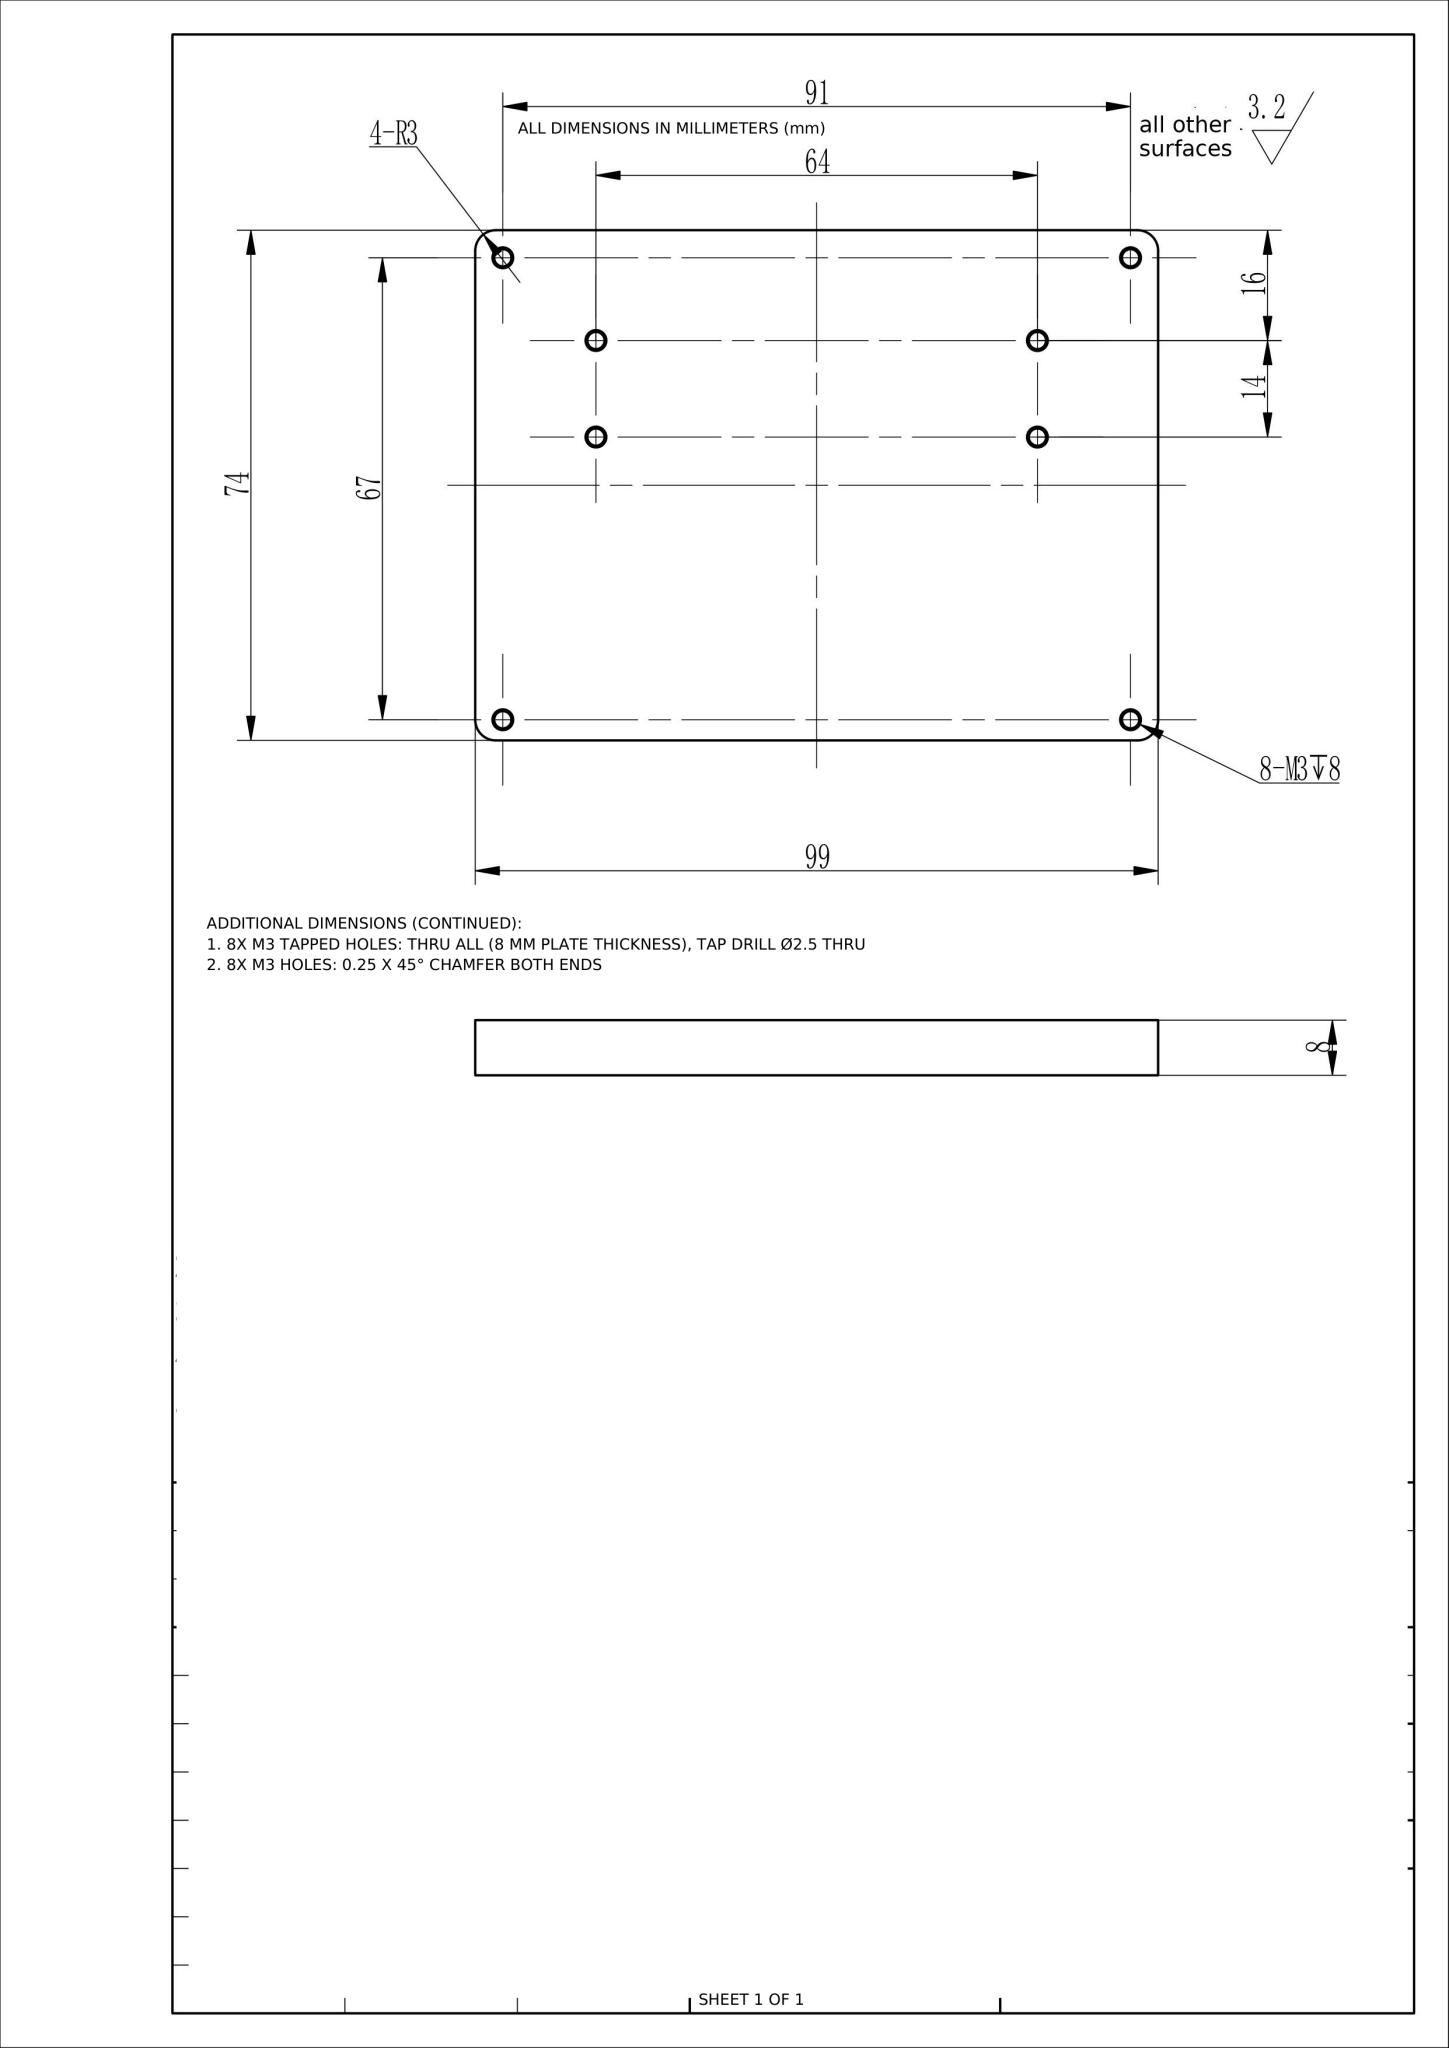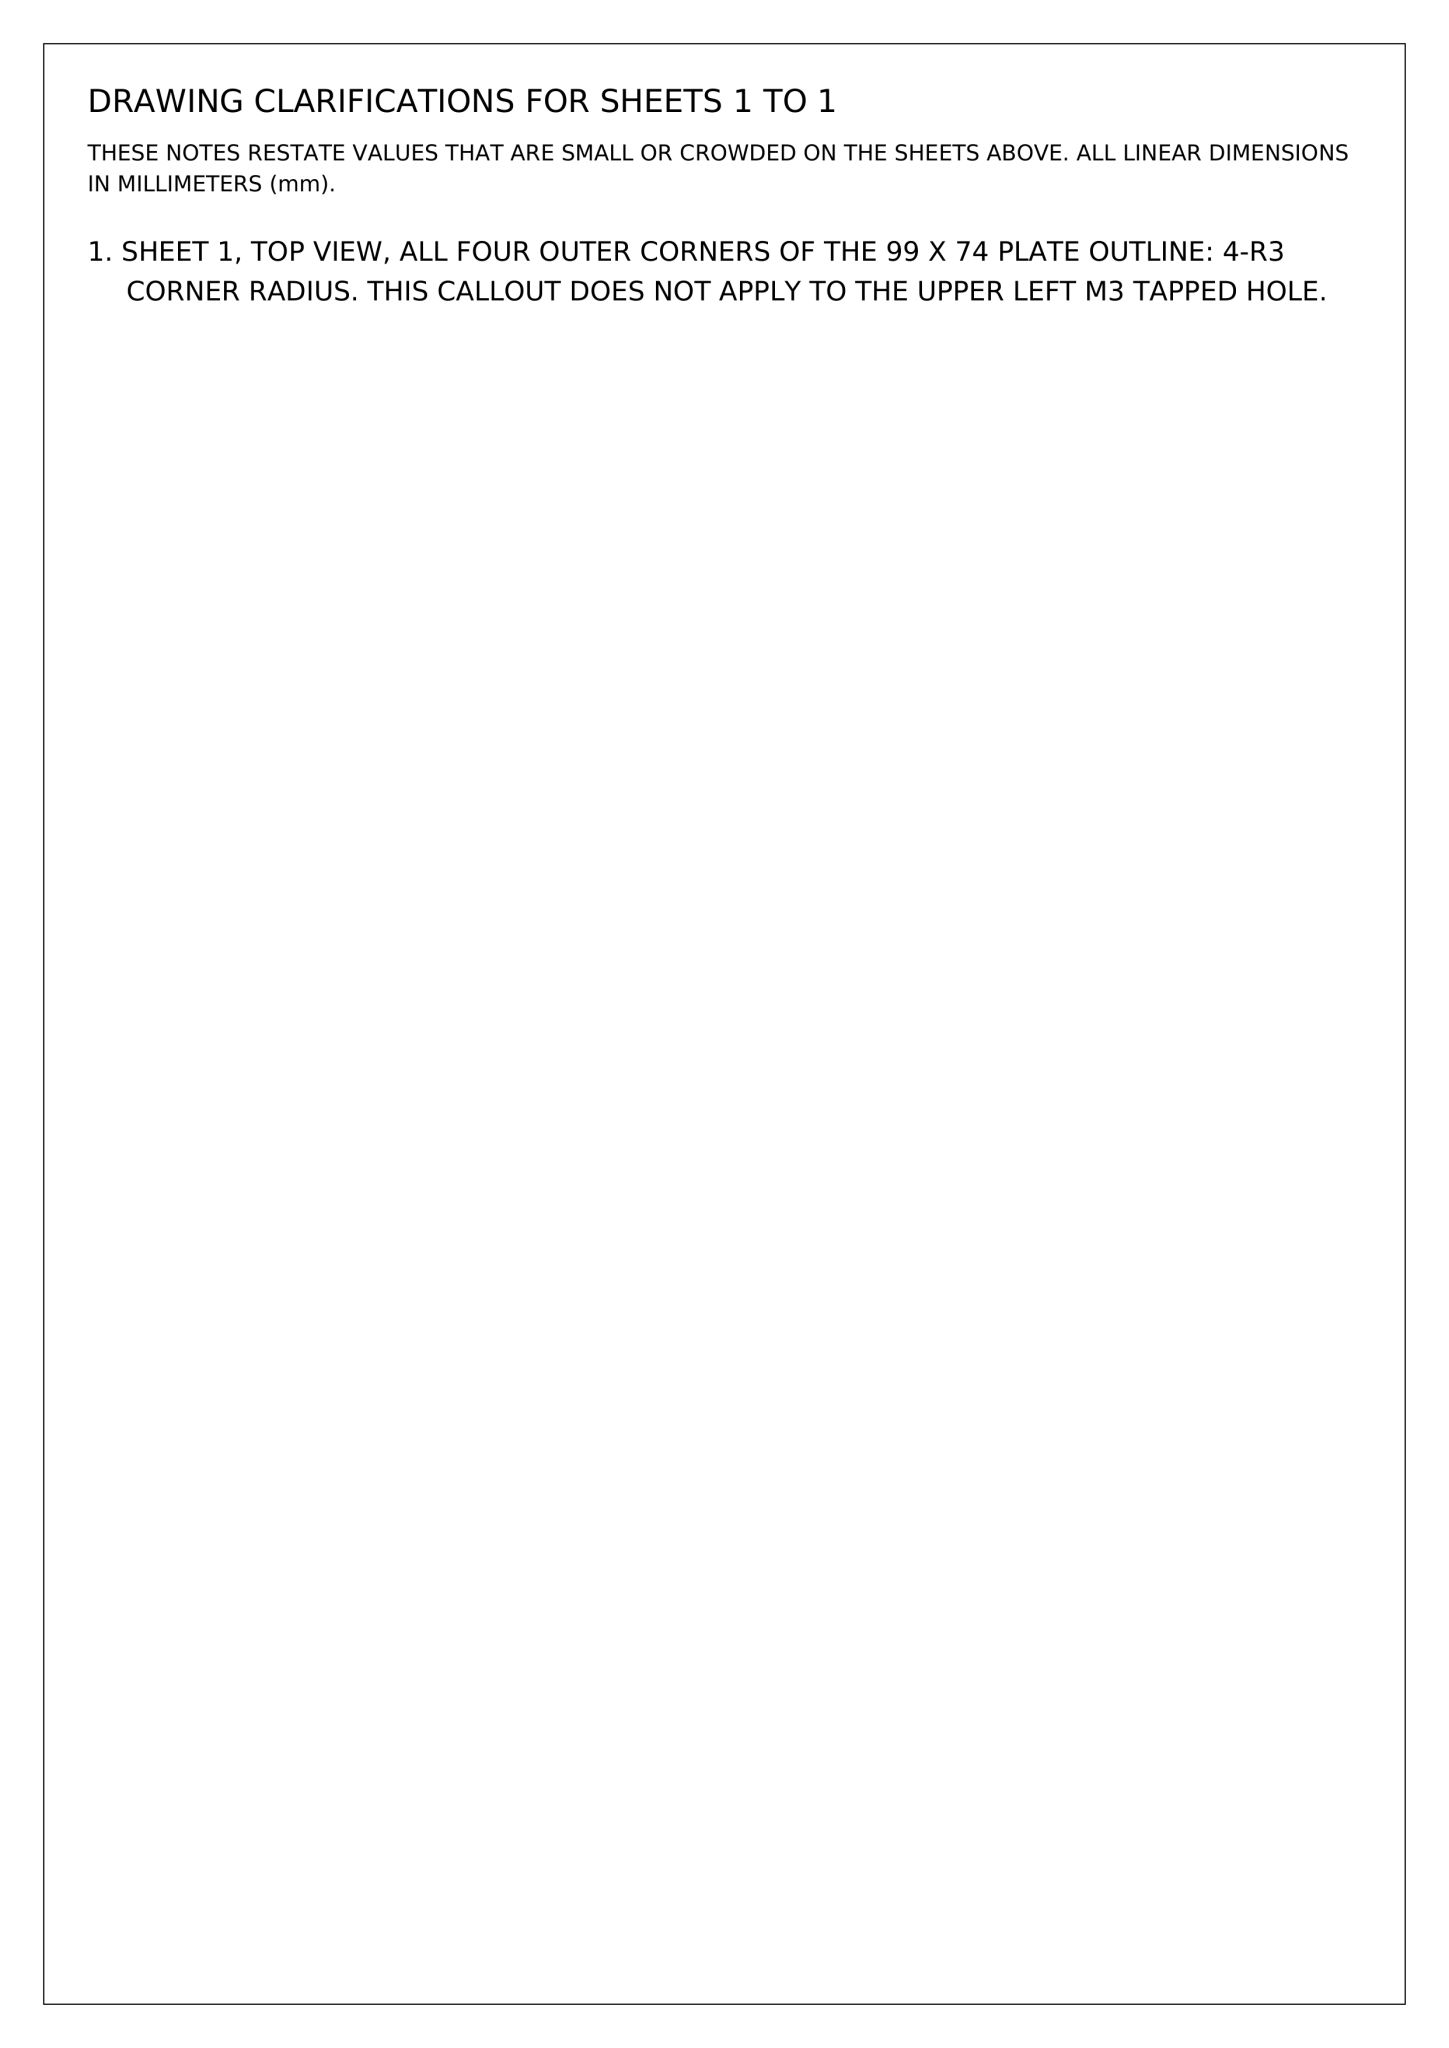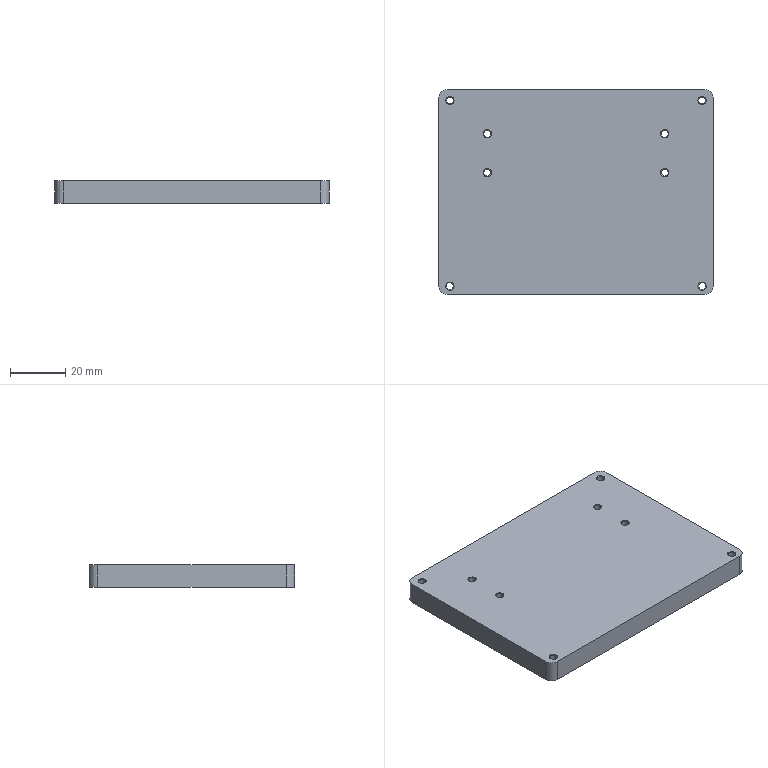Part | NX | mm | 1 solid | 34 faces | box 99 x 74 x 8 mm | volume 58228 mm3 | cone 16 | cylinder 12 | plane 6 | commonest cylinder face diameters 2.5 x8 6 x4
STEP:
#1=CARTESIAN_POINT('',(0.,0.,0.));
#2=DIRECTION('',(0.,0.,1.));
#3=DIRECTION('',(1.,0.,0.));
#4=AXIS2_PLACEMENT_3D('',#1,#2,#3);
#5=(LENGTH_UNIT()NAMED_UNIT(*)SI_UNIT(.MILLI.,.METRE.));
#6=UNCERTAINTY_MEASURE_WITH_UNIT(LENGTH_MEASURE(0.00002),#5,'','');
#7=(NAMED_UNIT(*)PLANE_ANGLE_UNIT()SI_UNIT($,.RADIAN.));
#8=PLANE_ANGLE_MEASURE_WITH_UNIT(PLANE_ANGLE_MEASURE(0.01745),#7);
#9=DIMENSIONAL_EXPONENTS(0.,0.,0.,0.,0.,0.,0.);
#10=(CONVERSION_BASED_UNIT('',#8)NAMED_UNIT(#9)PLANE_ANGLE_UNIT());
#11=(NAMED_UNIT(*)SI_UNIT($,.STERADIAN.)SOLID_ANGLE_UNIT());
#12=(GEOMETRIC_REPRESENTATION_CONTEXT(3)GLOBAL_UNCERTAINTY_ASSIGNED_CONTEXT((#6))GLOBAL_UNIT_ASSIGNED_CONTEXT((#5,#10,#11))REPRESENTATION_CONTEXT('',''));
#13=SHAPE_REPRESENTATION('',(#4),#12);
#14=CARTESIAN_POINT('',(-622.186,936.561,396.282));
#15=VERTEX_POINT('',#14);
#16=CARTESIAN_POINT('',(-622.186,1004.561,396.282));
#17=VERTEX_POINT('',#16);
#18=CARTESIAN_POINT('',(-622.186,933.561,396.282));
#19=DIRECTION('',(0.,1.,0.));
#20=VECTOR('',#19,1.);
#21=LINE('',#18,#20);
#22=EDGE_CURVE('',#15,#17,#21,.T.);
#23=ORIENTED_EDGE('',*,*,#22,.T.);
#24=CARTESIAN_POINT('',(-622.186,1004.561,388.282));
#25=VERTEX_POINT('',#24);
#26=CARTESIAN_POINT('',(-622.186,1004.561,388.282));
#27=DIRECTION('',(0.,0.,-1.));
#28=VECTOR('',#27,1.);
#29=LINE('',#26,#28);
#30=EDGE_CURVE('',#17,#25,#29,.T.);
#31=ORIENTED_EDGE('',*,*,#30,.T.);
#32=CARTESIAN_POINT('',(-622.186,936.561,388.282));
#33=VERTEX_POINT('',#32);
#34=CARTESIAN_POINT('',(-622.186,933.561,388.282));
#35=DIRECTION('',(0.,1.,0.));
#36=VECTOR('',#35,1.);
#37=LINE('',#34,#36);
#38=EDGE_CURVE('',#33,#25,#37,.T.);
#39=ORIENTED_EDGE('',*,*,#38,.F.);
#40=CARTESIAN_POINT('',(-622.186,936.561,388.282));
#41=DIRECTION('',(0.,0.,1.));
#42=VECTOR('',#41,1.);
#43=LINE('',#40,#42);
#44=EDGE_CURVE('',#33,#15,#43,.T.);
#45=ORIENTED_EDGE('',*,*,#44,.T.);
#46=EDGE_LOOP('',(#23,#31,#39,#45));
#47=FACE_OUTER_BOUND('',#46,.T.);
#48=CARTESIAN_POINT('',(-622.186,933.561,388.282));
#49=DIRECTION('',(1.,0.,0.));
#50=DIRECTION('',(0.,0.,-1.));
#51=AXIS2_PLACEMENT_3D('',#48,#49,#50);
#52=PLANE('',#51);
#53=ADVANCED_FACE('',(#47),#52,.F.);
#54=CARTESIAN_POINT('',(-619.186,1007.561,396.282));
#55=VERTEX_POINT('',#54);
#56=CARTESIAN_POINT('',(-526.186,1007.561,396.282));
#57=VERTEX_POINT('',#56);
#58=CARTESIAN_POINT('',(-622.186,1007.561,396.282));
#59=DIRECTION('',(1.,0.,0.));
#60=VECTOR('',#59,1.);
#61=LINE('',#58,#60);
#62=EDGE_CURVE('',#55,#57,#61,.T.);
#63=ORIENTED_EDGE('',*,*,#62,.T.);
#64=CARTESIAN_POINT('',(-526.186,1007.561,388.282));
#65=VERTEX_POINT('',#64);
#66=CARTESIAN_POINT('',(-526.186,1007.561,388.282));
#67=DIRECTION('',(0.,0.,-1.));
#68=VECTOR('',#67,1.);
#69=LINE('',#66,#68);
#70=EDGE_CURVE('',#57,#65,#69,.T.);
#71=ORIENTED_EDGE('',*,*,#70,.T.);
#72=CARTESIAN_POINT('',(-619.186,1007.561,388.282));
#73=VERTEX_POINT('',#72);
#74=CARTESIAN_POINT('',(-622.186,1007.561,388.282));
#75=DIRECTION('',(1.,0.,0.));
#76=VECTOR('',#75,1.);
#77=LINE('',#74,#76);
#78=EDGE_CURVE('',#73,#65,#77,.T.);
#79=ORIENTED_EDGE('',*,*,#78,.F.);
#80=CARTESIAN_POINT('',(-619.186,1007.561,388.282));
#81=DIRECTION('',(0.,0.,1.));
#82=VECTOR('',#81,1.);
#83=LINE('',#80,#82);
#84=EDGE_CURVE('',#73,#55,#83,.T.);
#85=ORIENTED_EDGE('',*,*,#84,.T.);
#86=EDGE_LOOP('',(#63,#71,#79,#85));
#87=FACE_OUTER_BOUND('',#86,.T.);
#88=CARTESIAN_POINT('',(-622.186,1007.561,388.282));
#89=DIRECTION('',(0.,-1.,0.));
#90=DIRECTION('',(0.,0.,-1.));
#91=AXIS2_PLACEMENT_3D('',#88,#89,#90);
#92=PLANE('',#91);
#93=ADVANCED_FACE('',(#87),#92,.F.);
#94=CARTESIAN_POINT('',(-523.186,1004.561,388.282));
#95=VERTEX_POINT('',#94);
#96=CARTESIAN_POINT('',(-523.186,936.561,388.282));
#97=VERTEX_POINT('',#96);
#98=CARTESIAN_POINT('',(-523.186,1007.561,388.282));
#99=DIRECTION('',(0.,-1.,0.));
#100=VECTOR('',#99,1.);
#101=LINE('',#98,#100);
#102=EDGE_CURVE('',#95,#97,#101,.T.);
#103=ORIENTED_EDGE('',*,*,#102,.F.);
#104=CARTESIAN_POINT('',(-523.186,1004.561,396.282));
#105=VERTEX_POINT('',#104);
#106=CARTESIAN_POINT('',(-523.186,1004.561,388.282));
#107=DIRECTION('',(0.,0.,1.));
#108=VECTOR('',#107,1.);
#109=LINE('',#106,#108);
#110=EDGE_CURVE('',#95,#105,#109,.T.);
#111=ORIENTED_EDGE('',*,*,#110,.T.);
#112=CARTESIAN_POINT('',(-523.186,936.561,396.282));
#113=VERTEX_POINT('',#112);
#114=CARTESIAN_POINT('',(-523.186,1007.561,396.282));
#115=DIRECTION('',(0.,-1.,0.));
#116=VECTOR('',#115,1.);
#117=LINE('',#114,#116);
#118=EDGE_CURVE('',#105,#113,#117,.T.);
#119=ORIENTED_EDGE('',*,*,#118,.T.);
#120=CARTESIAN_POINT('',(-523.186,936.561,388.282));
#121=DIRECTION('',(0.,0.,-1.));
#122=VECTOR('',#121,1.);
#123=LINE('',#120,#122);
#124=EDGE_CURVE('',#113,#97,#123,.T.);
#125=ORIENTED_EDGE('',*,*,#124,.T.);
#126=EDGE_LOOP('',(#103,#111,#119,#125));
#127=FACE_OUTER_BOUND('',#126,.T.);
#128=CARTESIAN_POINT('',(-523.186,1007.561,388.282));
#129=DIRECTION('',(-1.,0.,0.));
#130=DIRECTION('',(0.,0.,1.));
#131=AXIS2_PLACEMENT_3D('',#128,#129,#130);
#132=PLANE('',#131);
#133=ADVANCED_FACE('',(#127),#132,.F.);
#134=CARTESIAN_POINT('',(-526.186,933.561,388.282));
#135=VERTEX_POINT('',#134);
#136=CARTESIAN_POINT('',(-619.186,933.561,388.282));
#137=VERTEX_POINT('',#136);
#138=CARTESIAN_POINT('',(-523.186,933.561,388.282));
#139=DIRECTION('',(-1.,0.,0.));
#140=VECTOR('',#139,1.);
#141=LINE('',#138,#140);
#142=EDGE_CURVE('',#135,#137,#141,.T.);
#143=ORIENTED_EDGE('',*,*,#142,.F.);
#144=CARTESIAN_POINT('',(-526.186,933.561,396.282));
#145=VERTEX_POINT('',#144);
#146=CARTESIAN_POINT('',(-526.186,933.561,388.282));
#147=DIRECTION('',(0.,0.,1.));
#148=VECTOR('',#147,1.);
#149=LINE('',#146,#148);
#150=EDGE_CURVE('',#135,#145,#149,.T.);
#151=ORIENTED_EDGE('',*,*,#150,.T.);
#152=CARTESIAN_POINT('',(-619.186,933.561,396.282));
#153=VERTEX_POINT('',#152);
#154=CARTESIAN_POINT('',(-523.186,933.561,396.282));
#155=DIRECTION('',(-1.,0.,0.));
#156=VECTOR('',#155,1.);
#157=LINE('',#154,#156);
#158=EDGE_CURVE('',#145,#153,#157,.T.);
#159=ORIENTED_EDGE('',*,*,#158,.T.);
#160=CARTESIAN_POINT('',(-619.186,933.561,388.282));
#161=DIRECTION('',(0.,0.,-1.));
#162=VECTOR('',#161,1.);
#163=LINE('',#160,#162);
#164=EDGE_CURVE('',#153,#137,#163,.T.);
#165=ORIENTED_EDGE('',*,*,#164,.T.);
#166=EDGE_LOOP('',(#143,#151,#159,#165));
#167=FACE_OUTER_BOUND('',#166,.T.);
#168=CARTESIAN_POINT('',(-523.186,933.561,388.282));
#169=DIRECTION('',(0.,1.,0.));
#170=DIRECTION('',(0.,0.,1.));
#171=AXIS2_PLACEMENT_3D('',#168,#169,#170);
#172=PLANE('',#171);
#173=ADVANCED_FACE('',(#167),#172,.F.);
#174=CARTESIAN_POINT('',(-542.186,977.556,388.282));
#175=VERTEX_POINT('',#174);
#176=CARTESIAN_POINT('',(-540.686,977.556,388.282));
#177=DIRECTION('',(0.,0.,1.));
#178=DIRECTION('',(-1.,0.,0.));
#179=AXIS2_PLACEMENT_3D('',#176,#177,#178);
#180=CIRCLE('',#179,1.5);
#181=EDGE_CURVE('',#175,#175,#180,.T.);
#182=ORIENTED_EDGE('',*,*,#181,.T.);
#183=EDGE_LOOP('',(#182));
#184=FACE_BOUND('',#183,.T.);
#185=CARTESIAN_POINT('',(-542.186,991.556,388.282));
#186=VERTEX_POINT('',#185);
#187=CARTESIAN_POINT('',(-540.686,991.556,388.282));
#188=DIRECTION('',(0.,0.,1.));
#189=DIRECTION('',(-1.,0.,0.));
#190=AXIS2_PLACEMENT_3D('',#187,#188,#189);
#191=CIRCLE('',#190,1.5);
#192=EDGE_CURVE('',#186,#186,#191,.T.);
#193=ORIENTED_EDGE('',*,*,#192,.T.);
#194=EDGE_LOOP('',(#193));
#195=FACE_BOUND('',#194,.T.);
#196=CARTESIAN_POINT('',(-606.186,977.561,388.282));
#197=VERTEX_POINT('',#196);
#198=CARTESIAN_POINT('',(-604.686,977.561,388.282));
#199=DIRECTION('',(0.,0.,1.));
#200=DIRECTION('',(-1.,0.,0.));
#201=AXIS2_PLACEMENT_3D('',#198,#199,#200);
#202=CIRCLE('',#201,1.5);
#203=EDGE_CURVE('',#197,#197,#202,.T.);
#204=ORIENTED_EDGE('',*,*,#203,.T.);
#205=EDGE_LOOP('',(#204));
#206=FACE_BOUND('',#205,.T.);
#207=CARTESIAN_POINT('',(-606.186,991.561,388.282));
#208=VERTEX_POINT('',#207);
#209=CARTESIAN_POINT('',(-604.686,991.561,388.282));
#210=DIRECTION('',(0.,0.,1.));
#211=DIRECTION('',(-1.,0.,0.));
#212=AXIS2_PLACEMENT_3D('',#209,#210,#211);
#213=CIRCLE('',#212,1.5);
#214=EDGE_CURVE('',#208,#208,#213,.T.);
#215=ORIENTED_EDGE('',*,*,#214,.T.);
#216=EDGE_LOOP('',(#215));
#217=FACE_BOUND('',#216,.T.);
#218=CARTESIAN_POINT('',(-528.686,1003.561,388.282));
#219=VERTEX_POINT('',#218);
#220=CARTESIAN_POINT('',(-527.186,1003.561,388.282));
#221=DIRECTION('',(0.,0.,1.));
#222=DIRECTION('',(-1.,0.,0.));
#223=AXIS2_PLACEMENT_3D('',#220,#221,#222);
#224=CIRCLE('',#223,1.5);
#225=EDGE_CURVE('',#219,#219,#224,.T.);
#226=ORIENTED_EDGE('',*,*,#225,.T.);
#227=EDGE_LOOP('',(#226));
#228=FACE_BOUND('',#227,.T.);
#229=CARTESIAN_POINT('',(-528.686,936.561,388.282));
#230=VERTEX_POINT('',#229);
#231=CARTESIAN_POINT('',(-527.186,936.561,388.282));
#232=DIRECTION('',(0.,0.,1.));
#233=DIRECTION('',(-1.,0.,0.));
#234=AXIS2_PLACEMENT_3D('',#231,#232,#233);
#235=CIRCLE('',#234,1.5);
#236=EDGE_CURVE('',#230,#230,#235,.T.);
#237=ORIENTED_EDGE('',*,*,#236,.T.);
#238=EDGE_LOOP('',(#237));
#239=FACE_BOUND('',#238,.T.);
#240=CARTESIAN_POINT('',(-619.686,1003.561,388.282));
#241=VERTEX_POINT('',#240);
#242=CARTESIAN_POINT('',(-618.186,1003.561,388.282));
#243=DIRECTION('',(0.,0.,1.));
#244=DIRECTION('',(-1.,0.,0.));
#245=AXIS2_PLACEMENT_3D('',#242,#243,#244);
#246=CIRCLE('',#245,1.5);
#247=EDGE_CURVE('',#241,#241,#246,.T.);
#248=ORIENTED_EDGE('',*,*,#247,.T.);
#249=EDGE_LOOP('',(#248));
#250=FACE_BOUND('',#249,.T.);
#251=CARTESIAN_POINT('',(-619.686,936.561,388.282));
#252=VERTEX_POINT('',#251);
#253=CARTESIAN_POINT('',(-618.186,936.561,388.282));
#254=DIRECTION('',(0.,0.,1.));
#255=DIRECTION('',(-1.,0.,0.));
#256=AXIS2_PLACEMENT_3D('',#253,#254,#255);
#257=CIRCLE('',#256,1.5);
#258=EDGE_CURVE('',#252,#252,#257,.T.);
#259=ORIENTED_EDGE('',*,*,#258,.T.);
#260=EDGE_LOOP('',(#259));
#261=FACE_BOUND('',#260,.T.);
#262=ORIENTED_EDGE('',*,*,#78,.T.);
#263=CARTESIAN_POINT('',(-526.186,1004.561,388.282));
#264=DIRECTION('',(0.,0.,-1.));
#265=DIRECTION('',(-1.,0.,0.));
#266=AXIS2_PLACEMENT_3D('',#263,#264,#265);
#267=CIRCLE('',#266,3.);
#268=EDGE_CURVE('',#65,#95,#267,.T.);
#269=ORIENTED_EDGE('',*,*,#268,.T.);
#270=ORIENTED_EDGE('',*,*,#102,.T.);
#271=CARTESIAN_POINT('',(-526.186,936.561,388.282));
#272=DIRECTION('',(0.,0.,-1.));
#273=DIRECTION('',(-1.,0.,0.));
#274=AXIS2_PLACEMENT_3D('',#271,#272,#273);
#275=CIRCLE('',#274,3.);
#276=EDGE_CURVE('',#97,#135,#275,.T.);
#277=ORIENTED_EDGE('',*,*,#276,.T.);
#278=ORIENTED_EDGE('',*,*,#142,.T.);
#279=CARTESIAN_POINT('',(-619.186,936.561,388.282));
#280=DIRECTION('',(0.,0.,-1.));
#281=DIRECTION('',(-1.,0.,0.));
#282=AXIS2_PLACEMENT_3D('',#279,#280,#281);
#283=CIRCLE('',#282,3.);
#284=EDGE_CURVE('',#137,#33,#283,.T.);
#285=ORIENTED_EDGE('',*,*,#284,.T.);
#286=ORIENTED_EDGE('',*,*,#38,.T.);
#287=CARTESIAN_POINT('',(-619.186,1004.561,388.282));
#288=DIRECTION('',(0.,0.,-1.));
#289=DIRECTION('',(-1.,0.,0.));
#290=AXIS2_PLACEMENT_3D('',#287,#288,#289);
#291=CIRCLE('',#290,3.);
#292=EDGE_CURVE('',#25,#73,#291,.T.);
#293=ORIENTED_EDGE('',*,*,#292,.T.);
#294=EDGE_LOOP('',(#262,#269,#270,#277,#278,#285,#286,#293));
#295=FACE_BOUND('',#294,.T.);
#296=CARTESIAN_POINT('',(0.,0.,388.282));
#297=DIRECTION('',(0.,0.,-1.));
#298=DIRECTION('',(-1.,0.,0.));
#299=AXIS2_PLACEMENT_3D('',#296,#297,#298);
#300=PLANE('',#299);
#301=ADVANCED_FACE('',(#184,#195,#206,#217,#228,#239,#250,#261,#295),#300,.T.);
#302=CARTESIAN_POINT('',(-542.186,977.556,396.282));
#303=VERTEX_POINT('',#302);
#304=CARTESIAN_POINT('',(-540.686,977.556,396.282));
#305=DIRECTION('',(0.,0.,-1.));
#306=DIRECTION('',(-1.,0.,0.));
#307=AXIS2_PLACEMENT_3D('',#304,#305,#306);
#308=CIRCLE('',#307,1.5);
#309=EDGE_CURVE('',#303,#303,#308,.T.);
#310=ORIENTED_EDGE('',*,*,#309,.T.);
#311=EDGE_LOOP('',(#310));
#312=FACE_BOUND('',#311,.T.);
#313=CARTESIAN_POINT('',(-542.186,991.556,396.282));
#314=VERTEX_POINT('',#313);
#315=CARTESIAN_POINT('',(-540.686,991.556,396.282));
#316=DIRECTION('',(0.,0.,-1.));
#317=DIRECTION('',(-1.,0.,0.));
#318=AXIS2_PLACEMENT_3D('',#315,#316,#317);
#319=CIRCLE('',#318,1.5);
#320=EDGE_CURVE('',#314,#314,#319,.T.);
#321=ORIENTED_EDGE('',*,*,#320,.T.);
#322=EDGE_LOOP('',(#321));
#323=FACE_BOUND('',#322,.T.);
#324=CARTESIAN_POINT('',(-606.186,977.561,396.282));
#325=VERTEX_POINT('',#324);
#326=CARTESIAN_POINT('',(-604.686,977.561,396.282));
#327=DIRECTION('',(0.,0.,-1.));
#328=DIRECTION('',(-1.,0.,0.));
#329=AXIS2_PLACEMENT_3D('',#326,#327,#328);
#330=CIRCLE('',#329,1.5);
#331=EDGE_CURVE('',#325,#325,#330,.T.);
#332=ORIENTED_EDGE('',*,*,#331,.T.);
#333=EDGE_LOOP('',(#332));
#334=FACE_BOUND('',#333,.T.);
#335=CARTESIAN_POINT('',(-606.186,991.561,396.282));
#336=VERTEX_POINT('',#335);
#337=CARTESIAN_POINT('',(-604.686,991.561,396.282));
#338=DIRECTION('',(0.,0.,-1.));
#339=DIRECTION('',(-1.,0.,0.));
#340=AXIS2_PLACEMENT_3D('',#337,#338,#339);
#341=CIRCLE('',#340,1.5);
#342=EDGE_CURVE('',#336,#336,#341,.T.);
#343=ORIENTED_EDGE('',*,*,#342,.T.);
#344=EDGE_LOOP('',(#343));
#345=FACE_BOUND('',#344,.T.);
#346=CARTESIAN_POINT('',(-528.686,1003.561,396.282));
#347=VERTEX_POINT('',#346);
#348=CARTESIAN_POINT('',(-527.186,1003.561,396.282));
#349=DIRECTION('',(0.,0.,-1.));
#350=DIRECTION('',(-1.,0.,0.));
#351=AXIS2_PLACEMENT_3D('',#348,#349,#350);
#352=CIRCLE('',#351,1.5);
#353=EDGE_CURVE('',#347,#347,#352,.T.);
#354=ORIENTED_EDGE('',*,*,#353,.T.);
#355=EDGE_LOOP('',(#354));
#356=FACE_BOUND('',#355,.T.);
#357=CARTESIAN_POINT('',(-528.686,936.561,396.282));
#358=VERTEX_POINT('',#357);
#359=CARTESIAN_POINT('',(-527.186,936.561,396.282));
#360=DIRECTION('',(0.,0.,-1.));
#361=DIRECTION('',(-1.,0.,0.));
#362=AXIS2_PLACEMENT_3D('',#359,#360,#361);
#363=CIRCLE('',#362,1.5);
#364=EDGE_CURVE('',#358,#358,#363,.T.);
#365=ORIENTED_EDGE('',*,*,#364,.T.);
#366=EDGE_LOOP('',(#365));
#367=FACE_BOUND('',#366,.T.);
#368=CARTESIAN_POINT('',(-619.686,1003.561,396.282));
#369=VERTEX_POINT('',#368);
#370=CARTESIAN_POINT('',(-618.186,1003.561,396.282));
#371=DIRECTION('',(0.,0.,-1.));
#372=DIRECTION('',(-1.,0.,0.));
#373=AXIS2_PLACEMENT_3D('',#370,#371,#372);
#374=CIRCLE('',#373,1.5);
#375=EDGE_CURVE('',#369,#369,#374,.T.);
#376=ORIENTED_EDGE('',*,*,#375,.T.);
#377=EDGE_LOOP('',(#376));
#378=FACE_BOUND('',#377,.T.);
#379=CARTESIAN_POINT('',(-619.686,936.561,396.282));
#380=VERTEX_POINT('',#379);
#381=CARTESIAN_POINT('',(-618.186,936.561,396.282));
#382=DIRECTION('',(0.,0.,-1.));
#383=DIRECTION('',(-1.,0.,0.));
#384=AXIS2_PLACEMENT_3D('',#381,#382,#383);
#385=CIRCLE('',#384,1.5);
#386=EDGE_CURVE('',#380,#380,#385,.T.);
#387=ORIENTED_EDGE('',*,*,#386,.T.);
#388=EDGE_LOOP('',(#387));
#389=FACE_BOUND('',#388,.T.);
#390=ORIENTED_EDGE('',*,*,#118,.F.);
#391=CARTESIAN_POINT('',(-526.186,1004.561,396.282));
#392=DIRECTION('',(0.,0.,1.));
#393=DIRECTION('',(-1.,0.,0.));
#394=AXIS2_PLACEMENT_3D('',#391,#392,#393);
#395=CIRCLE('',#394,3.);
#396=EDGE_CURVE('',#105,#57,#395,.T.);
#397=ORIENTED_EDGE('',*,*,#396,.T.);
#398=ORIENTED_EDGE('',*,*,#62,.F.);
#399=CARTESIAN_POINT('',(-619.186,1004.561,396.282));
#400=DIRECTION('',(0.,0.,1.));
#401=DIRECTION('',(-1.,0.,0.));
#402=AXIS2_PLACEMENT_3D('',#399,#400,#401);
#403=CIRCLE('',#402,3.);
#404=EDGE_CURVE('',#55,#17,#403,.T.);
#405=ORIENTED_EDGE('',*,*,#404,.T.);
#406=ORIENTED_EDGE('',*,*,#22,.F.);
#407=CARTESIAN_POINT('',(-619.186,936.561,396.282));
#408=DIRECTION('',(0.,0.,1.));
#409=DIRECTION('',(-1.,0.,0.));
#410=AXIS2_PLACEMENT_3D('',#407,#408,#409);
#411=CIRCLE('',#410,3.);
#412=EDGE_CURVE('',#15,#153,#411,.T.);
#413=ORIENTED_EDGE('',*,*,#412,.T.);
#414=ORIENTED_EDGE('',*,*,#158,.F.);
#415=CARTESIAN_POINT('',(-526.186,936.561,396.282));
#416=DIRECTION('',(0.,0.,1.));
#417=DIRECTION('',(-1.,0.,0.));
#418=AXIS2_PLACEMENT_3D('',#415,#416,#417);
#419=CIRCLE('',#418,3.);
#420=EDGE_CURVE('',#145,#113,#419,.T.);
#421=ORIENTED_EDGE('',*,*,#420,.T.);
#422=EDGE_LOOP('',(#390,#397,#398,#405,#406,#413,#414,#421));
#423=FACE_BOUND('',#422,.T.);
#424=CARTESIAN_POINT('',(0.,0.,396.282));
#425=DIRECTION('',(0.,0.,-1.));
#426=DIRECTION('',(-1.,0.,0.));
#427=AXIS2_PLACEMENT_3D('',#424,#425,#426);
#428=PLANE('',#427);
#429=ADVANCED_FACE('',(#312,#323,#334,#345,#356,#367,#378,#389,#423),#428,.F.);
#430=ORIENTED_EDGE('',*,*,#268,.F.);
#431=ORIENTED_EDGE('',*,*,#70,.F.);
#432=ORIENTED_EDGE('',*,*,#396,.F.);
#433=ORIENTED_EDGE('',*,*,#110,.F.);
#434=EDGE_LOOP('',(#430,#431,#432,#433));
#435=FACE_OUTER_BOUND('',#434,.T.);
#436=CARTESIAN_POINT('',(-526.186,1004.561,388.282));
#437=DIRECTION('',(0.,0.,1.));
#438=DIRECTION('',(1.,0.,0.));
#439=AXIS2_PLACEMENT_3D('',#436,#437,#438);
#440=CYLINDRICAL_SURFACE('',#439,3.);
#441=ADVANCED_FACE('',(#435),#440,.T.);
#442=ORIENTED_EDGE('',*,*,#276,.F.);
#443=ORIENTED_EDGE('',*,*,#124,.F.);
#444=ORIENTED_EDGE('',*,*,#420,.F.);
#445=ORIENTED_EDGE('',*,*,#150,.F.);
#446=EDGE_LOOP('',(#442,#443,#444,#445));
#447=FACE_OUTER_BOUND('',#446,.T.);
#448=CARTESIAN_POINT('',(-526.186,936.561,388.282));
#449=DIRECTION('',(0.,0.,1.));
#450=DIRECTION('',(1.,0.,0.));
#451=AXIS2_PLACEMENT_3D('',#448,#449,#450);
#452=CYLINDRICAL_SURFACE('',#451,3.);
#453=ADVANCED_FACE('',(#447),#452,.T.);
#454=ORIENTED_EDGE('',*,*,#292,.F.);
#455=ORIENTED_EDGE('',*,*,#30,.F.);
#456=ORIENTED_EDGE('',*,*,#404,.F.);
#457=ORIENTED_EDGE('',*,*,#84,.F.);
#458=EDGE_LOOP('',(#454,#455,#456,#457));
#459=FACE_OUTER_BOUND('',#458,.T.);
#460=CARTESIAN_POINT('',(-619.186,1004.561,388.282));
#461=DIRECTION('',(0.,0.,1.));
#462=DIRECTION('',(1.,0.,0.));
#463=AXIS2_PLACEMENT_3D('',#460,#461,#462);
#464=CYLINDRICAL_SURFACE('',#463,3.);
#465=ADVANCED_FACE('',(#459),#464,.T.);
#466=ORIENTED_EDGE('',*,*,#284,.F.);
#467=ORIENTED_EDGE('',*,*,#164,.F.);
#468=ORIENTED_EDGE('',*,*,#412,.F.);
#469=ORIENTED_EDGE('',*,*,#44,.F.);
#470=EDGE_LOOP('',(#466,#467,#468,#469));
#471=FACE_OUTER_BOUND('',#470,.T.);
#472=CARTESIAN_POINT('',(-619.186,936.561,388.282));
#473=DIRECTION('',(0.,0.,1.));
#474=DIRECTION('',(1.,0.,0.));
#475=AXIS2_PLACEMENT_3D('',#472,#473,#474);
#476=CYLINDRICAL_SURFACE('',#475,3.);
#477=ADVANCED_FACE('',(#471),#476,.T.);
#478=CARTESIAN_POINT('',(-619.436,936.561,388.532));
#479=VERTEX_POINT('',#478);
#480=CARTESIAN_POINT('',(-618.186,936.561,388.532));
#481=DIRECTION('',(0.,0.,-1.));
#482=DIRECTION('',(-1.,0.,0.));
#483=AXIS2_PLACEMENT_3D('',#480,#481,#482);
#484=CIRCLE('',#483,1.25);
#485=EDGE_CURVE('',#479,#479,#484,.T.);
#486=ORIENTED_EDGE('',*,*,#485,.T.);
#487=EDGE_LOOP('',(#486));
#488=FACE_BOUND('',#487,.T.);
#489=CARTESIAN_POINT('',(-619.436,936.561,396.032));
#490=VERTEX_POINT('',#489);
#491=CARTESIAN_POINT('',(-618.186,936.561,396.032));
#492=DIRECTION('',(0.,0.,1.));
#493=DIRECTION('',(-1.,0.,0.));
#494=AXIS2_PLACEMENT_3D('',#491,#492,#493);
#495=CIRCLE('',#494,1.25);
#496=EDGE_CURVE('',#490,#490,#495,.T.);
#497=ORIENTED_EDGE('',*,*,#496,.T.);
#498=EDGE_LOOP('',(#497));
#499=FACE_BOUND('',#498,.T.);
#500=CARTESIAN_POINT('',(-618.186,936.561,396.282));
#501=DIRECTION('',(0.,0.,-1.));
#502=DIRECTION('',(-1.,0.,0.));
#503=AXIS2_PLACEMENT_3D('',#500,#501,#502);
#504=CYLINDRICAL_SURFACE('',#503,1.25);
#505=ADVANCED_FACE('',(#488,#499),#504,.F.);
#506=ORIENTED_EDGE('',*,*,#496,.F.);
#507=EDGE_LOOP('',(#506));
#508=FACE_BOUND('',#507,.T.);
#509=ORIENTED_EDGE('',*,*,#386,.F.);
#510=EDGE_LOOP('',(#509));
#511=FACE_BOUND('',#510,.T.);
#512=CARTESIAN_POINT('',(-618.186,936.561,396.282));
#513=DIRECTION('',(0.,0.,1.));
#514=DIRECTION('',(1.,0.,0.));
#515=AXIS2_PLACEMENT_3D('',#512,#513,#514);
#516=CONICAL_SURFACE('',#515,1.5,45.);
#517=ADVANCED_FACE('',(#508,#511),#516,.F.);
#518=ORIENTED_EDGE('',*,*,#258,.F.);
#519=EDGE_LOOP('',(#518));
#520=FACE_BOUND('',#519,.T.);
#521=ORIENTED_EDGE('',*,*,#485,.F.);
#522=EDGE_LOOP('',(#521));
#523=FACE_BOUND('',#522,.T.);
#524=CARTESIAN_POINT('',(-618.186,936.561,388.532));
#525=DIRECTION('',(0.,0.,-1.));
#526=DIRECTION('',(-1.,0.,-0.));
#527=AXIS2_PLACEMENT_3D('',#524,#525,#526);
#528=CONICAL_SURFACE('',#527,1.25,45.);
#529=ADVANCED_FACE('',(#520,#523),#528,.F.);
#530=CARTESIAN_POINT('',(-619.436,1003.561,388.532));
#531=VERTEX_POINT('',#530);
#532=CARTESIAN_POINT('',(-618.186,1003.561,388.532));
#533=DIRECTION('',(0.,0.,-1.));
#534=DIRECTION('',(-1.,0.,0.));
#535=AXIS2_PLACEMENT_3D('',#532,#533,#534);
#536=CIRCLE('',#535,1.25);
#537=EDGE_CURVE('',#531,#531,#536,.T.);
#538=ORIENTED_EDGE('',*,*,#537,.T.);
#539=EDGE_LOOP('',(#538));
#540=FACE_BOUND('',#539,.T.);
#541=CARTESIAN_POINT('',(-619.436,1003.561,396.032));
#542=VERTEX_POINT('',#541);
#543=CARTESIAN_POINT('',(-618.186,1003.561,396.032));
#544=DIRECTION('',(0.,0.,1.));
#545=DIRECTION('',(-1.,0.,0.));
#546=AXIS2_PLACEMENT_3D('',#543,#544,#545);
#547=CIRCLE('',#546,1.25);
#548=EDGE_CURVE('',#542,#542,#547,.T.);
#549=ORIENTED_EDGE('',*,*,#548,.T.);
#550=EDGE_LOOP('',(#549));
#551=FACE_BOUND('',#550,.T.);
#552=CARTESIAN_POINT('',(-618.186,1003.561,396.282));
#553=DIRECTION('',(0.,0.,-1.));
#554=DIRECTION('',(-1.,0.,0.));
#555=AXIS2_PLACEMENT_3D('',#552,#553,#554);
#556=CYLINDRICAL_SURFACE('',#555,1.25);
#557=ADVANCED_FACE('',(#540,#551),#556,.F.);
#558=ORIENTED_EDGE('',*,*,#548,.F.);
#559=EDGE_LOOP('',(#558));
#560=FACE_BOUND('',#559,.T.);
#561=ORIENTED_EDGE('',*,*,#375,.F.);
#562=EDGE_LOOP('',(#561));
#563=FACE_BOUND('',#562,.T.);
#564=CARTESIAN_POINT('',(-618.186,1003.561,396.282));
#565=DIRECTION('',(0.,0.,1.));
#566=DIRECTION('',(1.,0.,0.));
#567=AXIS2_PLACEMENT_3D('',#564,#565,#566);
#568=CONICAL_SURFACE('',#567,1.5,45.);
#569=ADVANCED_FACE('',(#560,#563),#568,.F.);
#570=ORIENTED_EDGE('',*,*,#247,.F.);
#571=EDGE_LOOP('',(#570));
#572=FACE_BOUND('',#571,.T.);
#573=ORIENTED_EDGE('',*,*,#537,.F.);
#574=EDGE_LOOP('',(#573));
#575=FACE_BOUND('',#574,.T.);
#576=CARTESIAN_POINT('',(-618.186,1003.561,388.532));
#577=DIRECTION('',(0.,0.,-1.));
#578=DIRECTION('',(-1.,0.,-0.));
#579=AXIS2_PLACEMENT_3D('',#576,#577,#578);
#580=CONICAL_SURFACE('',#579,1.25,45.);
#581=ADVANCED_FACE('',(#572,#575),#580,.F.);
#582=CARTESIAN_POINT('',(-528.436,936.561,388.532));
#583=VERTEX_POINT('',#582);
#584=CARTESIAN_POINT('',(-527.186,936.561,388.532));
#585=DIRECTION('',(0.,0.,-1.));
#586=DIRECTION('',(-1.,0.,0.));
#587=AXIS2_PLACEMENT_3D('',#584,#585,#586);
#588=CIRCLE('',#587,1.25);
#589=EDGE_CURVE('',#583,#583,#588,.T.);
#590=ORIENTED_EDGE('',*,*,#589,.T.);
#591=EDGE_LOOP('',(#590));
#592=FACE_BOUND('',#591,.T.);
#593=CARTESIAN_POINT('',(-528.436,936.561,396.032));
#594=VERTEX_POINT('',#593);
#595=CARTESIAN_POINT('',(-527.186,936.561,396.032));
#596=DIRECTION('',(0.,0.,1.));
#597=DIRECTION('',(-1.,0.,0.));
#598=AXIS2_PLACEMENT_3D('',#595,#596,#597);
#599=CIRCLE('',#598,1.25);
#600=EDGE_CURVE('',#594,#594,#599,.T.);
#601=ORIENTED_EDGE('',*,*,#600,.T.);
#602=EDGE_LOOP('',(#601));
#603=FACE_BOUND('',#602,.T.);
#604=CARTESIAN_POINT('',(-527.186,936.561,396.282));
#605=DIRECTION('',(0.,0.,-1.));
#606=DIRECTION('',(-1.,0.,0.));
#607=AXIS2_PLACEMENT_3D('',#604,#605,#606);
#608=CYLINDRICAL_SURFACE('',#607,1.25);
#609=ADVANCED_FACE('',(#592,#603),#608,.F.);
#610=ORIENTED_EDGE('',*,*,#600,.F.);
#611=EDGE_LOOP('',(#610));
#612=FACE_BOUND('',#611,.T.);
#613=ORIENTED_EDGE('',*,*,#364,.F.);
#614=EDGE_LOOP('',(#613));
#615=FACE_BOUND('',#614,.T.);
#616=CARTESIAN_POINT('',(-527.186,936.561,396.282));
#617=DIRECTION('',(0.,0.,1.));
#618=DIRECTION('',(1.,0.,0.));
#619=AXIS2_PLACEMENT_3D('',#616,#617,#618);
#620=CONICAL_SURFACE('',#619,1.5,45.);
#621=ADVANCED_FACE('',(#612,#615),#620,.F.);
#622=ORIENTED_EDGE('',*,*,#236,.F.);
#623=EDGE_LOOP('',(#622));
#624=FACE_BOUND('',#623,.T.);
#625=ORIENTED_EDGE('',*,*,#589,.F.);
#626=EDGE_LOOP('',(#625));
#627=FACE_BOUND('',#626,.T.);
#628=CARTESIAN_POINT('',(-527.186,936.561,388.532));
#629=DIRECTION('',(0.,0.,-1.));
#630=DIRECTION('',(-1.,0.,-0.));
#631=AXIS2_PLACEMENT_3D('',#628,#629,#630);
#632=CONICAL_SURFACE('',#631,1.25,45.);
#633=ADVANCED_FACE('',(#624,#627),#632,.F.);
#634=CARTESIAN_POINT('',(-528.436,1003.561,388.532));
#635=VERTEX_POINT('',#634);
#636=CARTESIAN_POINT('',(-527.186,1003.561,388.532));
#637=DIRECTION('',(0.,0.,-1.));
#638=DIRECTION('',(-1.,0.,0.));
#639=AXIS2_PLACEMENT_3D('',#636,#637,#638);
#640=CIRCLE('',#639,1.25);
#641=EDGE_CURVE('',#635,#635,#640,.T.);
#642=ORIENTED_EDGE('',*,*,#641,.T.);
#643=EDGE_LOOP('',(#642));
#644=FACE_BOUND('',#643,.T.);
#645=CARTESIAN_POINT('',(-528.436,1003.561,396.032));
#646=VERTEX_POINT('',#645);
#647=CARTESIAN_POINT('',(-527.186,1003.561,396.032));
#648=DIRECTION('',(0.,0.,1.));
#649=DIRECTION('',(-1.,0.,0.));
#650=AXIS2_PLACEMENT_3D('',#647,#648,#649);
#651=CIRCLE('',#650,1.25);
#652=EDGE_CURVE('',#646,#646,#651,.T.);
#653=ORIENTED_EDGE('',*,*,#652,.T.);
#654=EDGE_LOOP('',(#653));
#655=FACE_BOUND('',#654,.T.);
#656=CARTESIAN_POINT('',(-527.186,1003.561,396.282));
#657=DIRECTION('',(0.,0.,-1.));
#658=DIRECTION('',(-1.,0.,0.));
#659=AXIS2_PLACEMENT_3D('',#656,#657,#658);
#660=CYLINDRICAL_SURFACE('',#659,1.25);
#661=ADVANCED_FACE('',(#644,#655),#660,.F.);
#662=ORIENTED_EDGE('',*,*,#652,.F.);
#663=EDGE_LOOP('',(#662));
#664=FACE_BOUND('',#663,.T.);
#665=ORIENTED_EDGE('',*,*,#353,.F.);
#666=EDGE_LOOP('',(#665));
#667=FACE_BOUND('',#666,.T.);
#668=CARTESIAN_POINT('',(-527.186,1003.561,396.282));
#669=DIRECTION('',(0.,0.,1.));
#670=DIRECTION('',(1.,0.,0.));
#671=AXIS2_PLACEMENT_3D('',#668,#669,#670);
#672=CONICAL_SURFACE('',#671,1.5,45.);
#673=ADVANCED_FACE('',(#664,#667),#672,.F.);
#674=ORIENTED_EDGE('',*,*,#225,.F.);
#675=EDGE_LOOP('',(#674));
#676=FACE_BOUND('',#675,.T.);
#677=ORIENTED_EDGE('',*,*,#641,.F.);
#678=EDGE_LOOP('',(#677));
#679=FACE_BOUND('',#678,.T.);
#680=CARTESIAN_POINT('',(-527.186,1003.561,388.532));
#681=DIRECTION('',(0.,0.,-1.));
#682=DIRECTION('',(-1.,0.,-0.));
#683=AXIS2_PLACEMENT_3D('',#680,#681,#682);
#684=CONICAL_SURFACE('',#683,1.25,45.);
#685=ADVANCED_FACE('',(#676,#679),#684,.F.);
#686=CARTESIAN_POINT('',(-605.936,991.561,388.532));
#687=VERTEX_POINT('',#686);
#688=CARTESIAN_POINT('',(-604.686,991.561,388.532));
#689=DIRECTION('',(0.,0.,-1.));
#690=DIRECTION('',(-1.,0.,0.));
#691=AXIS2_PLACEMENT_3D('',#688,#689,#690);
#692=CIRCLE('',#691,1.25);
#693=EDGE_CURVE('',#687,#687,#692,.T.);
#694=ORIENTED_EDGE('',*,*,#693,.T.);
#695=EDGE_LOOP('',(#694));
#696=FACE_BOUND('',#695,.T.);
#697=CARTESIAN_POINT('',(-605.936,991.561,396.032));
#698=VERTEX_POINT('',#697);
#699=CARTESIAN_POINT('',(-604.686,991.561,396.032));
#700=DIRECTION('',(0.,0.,1.));
#701=DIRECTION('',(-1.,0.,0.));
#702=AXIS2_PLACEMENT_3D('',#699,#700,#701);
#703=CIRCLE('',#702,1.25);
#704=EDGE_CURVE('',#698,#698,#703,.T.);
#705=ORIENTED_EDGE('',*,*,#704,.T.);
#706=EDGE_LOOP('',(#705));
#707=FACE_BOUND('',#706,.T.);
#708=CARTESIAN_POINT('',(-604.686,991.561,396.282));
#709=DIRECTION('',(0.,0.,-1.));
#710=DIRECTION('',(-1.,0.,0.));
#711=AXIS2_PLACEMENT_3D('',#708,#709,#710);
#712=CYLINDRICAL_SURFACE('',#711,1.25);
#713=ADVANCED_FACE('',(#696,#707),#712,.F.);
#714=ORIENTED_EDGE('',*,*,#704,.F.);
#715=EDGE_LOOP('',(#714));
#716=FACE_BOUND('',#715,.T.);
#717=ORIENTED_EDGE('',*,*,#342,.F.);
#718=EDGE_LOOP('',(#717));
#719=FACE_BOUND('',#718,.T.);
#720=CARTESIAN_POINT('',(-604.686,991.561,396.282));
#721=DIRECTION('',(0.,0.,1.));
#722=DIRECTION('',(1.,0.,0.));
#723=AXIS2_PLACEMENT_3D('',#720,#721,#722);
#724=CONICAL_SURFACE('',#723,1.5,45.);
#725=ADVANCED_FACE('',(#716,#719),#724,.F.);
#726=ORIENTED_EDGE('',*,*,#214,.F.);
#727=EDGE_LOOP('',(#726));
#728=FACE_BOUND('',#727,.T.);
#729=ORIENTED_EDGE('',*,*,#693,.F.);
#730=EDGE_LOOP('',(#729));
#731=FACE_BOUND('',#730,.T.);
#732=CARTESIAN_POINT('',(-604.686,991.561,388.532));
#733=DIRECTION('',(0.,0.,-1.));
#734=DIRECTION('',(-1.,0.,-0.));
#735=AXIS2_PLACEMENT_3D('',#732,#733,#734);
#736=CONICAL_SURFACE('',#735,1.25,45.);
#737=ADVANCED_FACE('',(#728,#731),#736,.F.);
#738=CARTESIAN_POINT('',(-605.936,977.561,388.532));
#739=VERTEX_POINT('',#738);
#740=CARTESIAN_POINT('',(-604.686,977.561,388.532));
#741=DIRECTION('',(0.,0.,-1.));
#742=DIRECTION('',(-1.,0.,0.));
#743=AXIS2_PLACEMENT_3D('',#740,#741,#742);
#744=CIRCLE('',#743,1.25);
#745=EDGE_CURVE('',#739,#739,#744,.T.);
#746=ORIENTED_EDGE('',*,*,#745,.T.);
#747=EDGE_LOOP('',(#746));
#748=FACE_BOUND('',#747,.T.);
#749=CARTESIAN_POINT('',(-605.936,977.561,396.032));
#750=VERTEX_POINT('',#749);
#751=CARTESIAN_POINT('',(-604.686,977.561,396.032));
#752=DIRECTION('',(0.,0.,1.));
#753=DIRECTION('',(-1.,0.,0.));
#754=AXIS2_PLACEMENT_3D('',#751,#752,#753);
#755=CIRCLE('',#754,1.25);
#756=EDGE_CURVE('',#750,#750,#755,.T.);
#757=ORIENTED_EDGE('',*,*,#756,.T.);
#758=EDGE_LOOP('',(#757));
#759=FACE_BOUND('',#758,.T.);
#760=CARTESIAN_POINT('',(-604.686,977.561,396.282));
#761=DIRECTION('',(0.,0.,-1.));
#762=DIRECTION('',(-1.,0.,0.));
#763=AXIS2_PLACEMENT_3D('',#760,#761,#762);
#764=CYLINDRICAL_SURFACE('',#763,1.25);
#765=ADVANCED_FACE('',(#748,#759),#764,.F.);
#766=ORIENTED_EDGE('',*,*,#756,.F.);
#767=EDGE_LOOP('',(#766));
#768=FACE_BOUND('',#767,.T.);
#769=ORIENTED_EDGE('',*,*,#331,.F.);
#770=EDGE_LOOP('',(#769));
#771=FACE_BOUND('',#770,.T.);
#772=CARTESIAN_POINT('',(-604.686,977.561,396.282));
#773=DIRECTION('',(0.,0.,1.));
#774=DIRECTION('',(1.,0.,0.));
#775=AXIS2_PLACEMENT_3D('',#772,#773,#774);
#776=CONICAL_SURFACE('',#775,1.5,45.);
#777=ADVANCED_FACE('',(#768,#771),#776,.F.);
#778=ORIENTED_EDGE('',*,*,#203,.F.);
#779=EDGE_LOOP('',(#778));
#780=FACE_BOUND('',#779,.T.);
#781=ORIENTED_EDGE('',*,*,#745,.F.);
#782=EDGE_LOOP('',(#781));
#783=FACE_BOUND('',#782,.T.);
#784=CARTESIAN_POINT('',(-604.686,977.561,388.532));
#785=DIRECTION('',(0.,0.,-1.));
#786=DIRECTION('',(-1.,0.,-0.));
#787=AXIS2_PLACEMENT_3D('',#784,#785,#786);
#788=CONICAL_SURFACE('',#787,1.25,45.);
#789=ADVANCED_FACE('',(#780,#783),#788,.F.);
#790=CARTESIAN_POINT('',(-541.936,991.556,388.532));
#791=VERTEX_POINT('',#790);
#792=CARTESIAN_POINT('',(-540.686,991.556,388.532));
#793=DIRECTION('',(0.,0.,-1.));
#794=DIRECTION('',(-1.,0.,0.));
#795=AXIS2_PLACEMENT_3D('',#792,#793,#794);
#796=CIRCLE('',#795,1.25);
#797=EDGE_CURVE('',#791,#791,#796,.T.);
#798=ORIENTED_EDGE('',*,*,#797,.T.);
#799=EDGE_LOOP('',(#798));
#800=FACE_BOUND('',#799,.T.);
#801=CARTESIAN_POINT('',(-541.936,991.556,396.032));
#802=VERTEX_POINT('',#801);
#803=CARTESIAN_POINT('',(-540.686,991.556,396.032));
#804=DIRECTION('',(0.,0.,1.));
#805=DIRECTION('',(-1.,0.,0.));
#806=AXIS2_PLACEMENT_3D('',#803,#804,#805);
#807=CIRCLE('',#806,1.25);
#808=EDGE_CURVE('',#802,#802,#807,.T.);
#809=ORIENTED_EDGE('',*,*,#808,.T.);
#810=EDGE_LOOP('',(#809));
#811=FACE_BOUND('',#810,.T.);
#812=CARTESIAN_POINT('',(-540.686,991.556,396.282));
#813=DIRECTION('',(0.,0.,-1.));
#814=DIRECTION('',(-1.,0.,0.));
#815=AXIS2_PLACEMENT_3D('',#812,#813,#814);
#816=CYLINDRICAL_SURFACE('',#815,1.25);
#817=ADVANCED_FACE('',(#800,#811),#816,.F.);
#818=ORIENTED_EDGE('',*,*,#808,.F.);
#819=EDGE_LOOP('',(#818));
#820=FACE_BOUND('',#819,.T.);
#821=ORIENTED_EDGE('',*,*,#320,.F.);
#822=EDGE_LOOP('',(#821));
#823=FACE_BOUND('',#822,.T.);
#824=CARTESIAN_POINT('',(-540.686,991.556,396.282));
#825=DIRECTION('',(0.,0.,1.));
#826=DIRECTION('',(1.,0.,0.));
#827=AXIS2_PLACEMENT_3D('',#824,#825,#826);
#828=CONICAL_SURFACE('',#827,1.5,45.);
#829=ADVANCED_FACE('',(#820,#823),#828,.F.);
#830=ORIENTED_EDGE('',*,*,#192,.F.);
#831=EDGE_LOOP('',(#830));
#832=FACE_BOUND('',#831,.T.);
#833=ORIENTED_EDGE('',*,*,#797,.F.);
#834=EDGE_LOOP('',(#833));
#835=FACE_BOUND('',#834,.T.);
#836=CARTESIAN_POINT('',(-540.686,991.556,388.532));
#837=DIRECTION('',(0.,0.,-1.));
#838=DIRECTION('',(-1.,0.,-0.));
#839=AXIS2_PLACEMENT_3D('',#836,#837,#838);
#840=CONICAL_SURFACE('',#839,1.25,45.);
#841=ADVANCED_FACE('',(#832,#835),#840,.F.);
#842=CARTESIAN_POINT('',(-541.936,977.556,388.532));
#843=VERTEX_POINT('',#842);
#844=CARTESIAN_POINT('',(-540.686,977.556,388.532));
#845=DIRECTION('',(0.,0.,-1.));
#846=DIRECTION('',(-1.,0.,0.));
#847=AXIS2_PLACEMENT_3D('',#844,#845,#846);
#848=CIRCLE('',#847,1.25);
#849=EDGE_CURVE('',#843,#843,#848,.T.);
#850=ORIENTED_EDGE('',*,*,#849,.T.);
#851=EDGE_LOOP('',(#850));
#852=FACE_BOUND('',#851,.T.);
#853=CARTESIAN_POINT('',(-541.936,977.556,396.032));
#854=VERTEX_POINT('',#853);
#855=CARTESIAN_POINT('',(-540.686,977.556,396.032));
#856=DIRECTION('',(0.,0.,1.));
#857=DIRECTION('',(-1.,0.,0.));
#858=AXIS2_PLACEMENT_3D('',#855,#856,#857);
#859=CIRCLE('',#858,1.25);
#860=EDGE_CURVE('',#854,#854,#859,.T.);
#861=ORIENTED_EDGE('',*,*,#860,.T.);
#862=EDGE_LOOP('',(#861));
#863=FACE_BOUND('',#862,.T.);
#864=CARTESIAN_POINT('',(-540.686,977.556,396.282));
#865=DIRECTION('',(0.,0.,-1.));
#866=DIRECTION('',(-1.,0.,0.));
#867=AXIS2_PLACEMENT_3D('',#864,#865,#866);
#868=CYLINDRICAL_SURFACE('',#867,1.25);
#869=ADVANCED_FACE('',(#852,#863),#868,.F.);
#870=ORIENTED_EDGE('',*,*,#860,.F.);
#871=EDGE_LOOP('',(#870));
#872=FACE_BOUND('',#871,.T.);
#873=ORIENTED_EDGE('',*,*,#309,.F.);
#874=EDGE_LOOP('',(#873));
#875=FACE_BOUND('',#874,.T.);
#876=CARTESIAN_POINT('',(-540.686,977.556,396.282));
#877=DIRECTION('',(0.,0.,1.));
#878=DIRECTION('',(1.,0.,0.));
#879=AXIS2_PLACEMENT_3D('',#876,#877,#878);
#880=CONICAL_SURFACE('',#879,1.5,45.);
#881=ADVANCED_FACE('',(#872,#875),#880,.F.);
#882=ORIENTED_EDGE('',*,*,#181,.F.);
#883=EDGE_LOOP('',(#882));
#884=FACE_BOUND('',#883,.T.);
#885=ORIENTED_EDGE('',*,*,#849,.F.);
#886=EDGE_LOOP('',(#885));
#887=FACE_BOUND('',#886,.T.);
#888=CARTESIAN_POINT('',(-540.686,977.556,388.532));
#889=DIRECTION('',(0.,0.,-1.));
#890=DIRECTION('',(-1.,0.,-0.));
#891=AXIS2_PLACEMENT_3D('',#888,#889,#890);
#892=CONICAL_SURFACE('',#891,1.25,45.);
#893=ADVANCED_FACE('',(#884,#887),#892,.F.);
#894=CLOSED_SHELL('',(#53,#93,#133,#173,#301,#429,#441,#453,#465,#477,#505,#517,#529,#557,#569,#581,#609,#621,#633,#661,#673,#685,#713,#725,#737,#765,#777,#789,#817,#829,#841,#869,#881,#893));
#895=MANIFOLD_SOLID_BREP('',#894);
#896=ADVANCED_BREP_SHAPE_REPRESENTATION('',(#895),#12);
#897=SHAPE_REPRESENTATION_RELATIONSHIP('','',#13,#896);
#898=PRESENTATION_LAYER_ASSIGNMENT('','',(#895));
#899=COLOUR_RGB('',1.,0.6,0.);
#900=FILL_AREA_STYLE_COLOUR('',#899);
#901=FILL_AREA_STYLE('',(#900));
#902=SURFACE_STYLE_FILL_AREA(#901);
#903=SURFACE_SIDE_STYLE('',(#902));
#904=SURFACE_STYLE_USAGE(.BOTH.,#903);
#905=PRESENTATION_STYLE_ASSIGNMENT((#904));
#906=STYLED_ITEM('',(#905),#895);
#907=MECHANICAL_DESIGN_GEOMETRIC_PRESENTATION_REPRESENTATION('',(#906),#12);